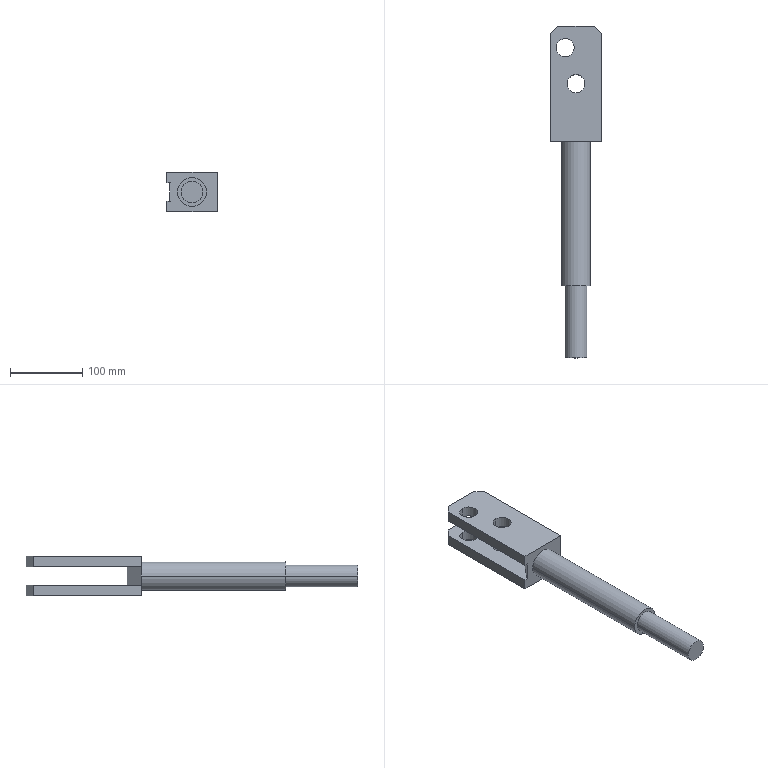Component | SolidWorks | Right-handTieRod1-1 | 1 solid | 30 faces | box 70 x 460 x 55 mm | volume 654381 mm3 | plane 18 | cylinder 12 | commonest cylinder face diameters 25 x8 30 x2 40 x2 | material N/A
build123d program:
from build123d import *

# Parameters (mm, degrees)
BOSS_EXTRUDE1_DEPTH      = 35
SKETCH2_R                = 12.5
CUT_EXTRUDE1_DEPTH       = 60
CHAMFER1_SIZE            = 10
SKETCH3_R                = 20
BOSS_EXTRUDE2_DEPTH      = 300
CHAMFER2_SIZE            = 5
CHAMFER2_SIZE2           = 8.66
SKETCH4_OUTSIDE_W        = 165.706
SKETCH4_OUTSIDE_H        = 150.706
SKETCH4_OUTSIDE_R        = 15
CUT_EXTRUDE2_DEPTH       = 100
CLEVISRELIEF_CRANK_DEPTH = 12.5


with BuildPart() as part:
    # Sketch1 → Boss-Extrude1 (new, symmetric)
    with BuildSketch(Plane(origin=(0, 0, 0), x_dir=(0, 0, -1), z_dir=(1, 0, 0))):
        Polygon((80, 12.5), (-60, 12.5), (-60, -12.5), (80, -12.5), (80, -27.5), (-80, -27.5), (-80, 27.5), (80, 27.5), align=None)
    extrude(amount=BOSS_EXTRUDE1_DEPTH, both=True)

    # Sketch2 → Cut-Extrude1 (cut)
    with BuildSketch(Plane.XZ.offset(27.5)):
        with Locations(Location((-15, -50, 0), (0, 0, 270))):
            Circle(SKETCH2_R)
        with Locations(Location((0, 0, 0), (0, 0, 270))):
            Circle(SKETCH2_R)
    extrude(amount=-CUT_EXTRUDE1_DEPTH, mode=Mode.SUBTRACT)

    # Chamfer1
    chamfer1_edges = [part.edges().sort_by_distance(p)[0] for p in [
        (-35, 20, -80),
        (35, -20, -80),
        (35, 20, -80),
        (-35, -20, -80),
    ]]
    chamfer(chamfer1_edges, length=CHAMFER1_SIZE)

    # Sketch3 → Boss-Extrude2 (add)
    with BuildSketch(Plane.XY.offset(80)):
        Circle(SKETCH3_R)
    extrude(amount=BOSS_EXTRUDE2_DEPTH)

    # Chamfer2
    chamfer2_edges = [part.edges().sort_by_distance(p)[0] for p in [
        (-35, 0, 60),
    ]]
    chamfer2_side = [part.faces().sort_by_distance(p)[0] for p in [
        (-35, 14.098, -5),
    ]]
    chamfer(chamfer2_edges, length=CHAMFER2_SIZE, length2=CHAMFER2_SIZE2, reference=chamfer2_side[0])

    # Sketch4 outside → Cut-Extrude2 (cut)
    with BuildSketch(Plane.XY.offset(380)):
        Rectangle(SKETCH4_OUTSIDE_W, SKETCH4_OUTSIDE_H)
        Circle(SKETCH4_OUTSIDE_R, mode=Mode.SUBTRACT)
    extrude(amount=-CUT_EXTRUDE2_DEPTH, mode=Mode.SUBTRACT)

    # ClevisRelief_Sketch → ClevisRelief_Crank (cut, symmetric)
    with BuildSketch(Plane(origin=(0, 0, 0), x_dir=(1, 0, 0), z_dir=(0, 1, 0))):
        Polygon((-11.942, -57), (-33.339, -83), (-40, -83), (-40, -57), align=None)
    extrude(amount=CLEVISRELIEF_CRANK_DEPTH, both=True, mode=Mode.SUBTRACT)


solid = part.part

# Placed as in the assembly
solid = solid.moved(Location((69.344, 1052.787, 17), (90, 0, 0)))
STEP:
#1=COLOUR_RGB('',0.7922,0.8196,0.9333);
#2=FILL_AREA_STYLE_COLOUR('',#1);
#3=FILL_AREA_STYLE('',(#2));
#4=SURFACE_STYLE_FILL_AREA(#3);
#5=SURFACE_SIDE_STYLE('',(#4));
#6=SURFACE_STYLE_USAGE(.BOTH.,#5);
#7=PRESENTATION_STYLE_ASSIGNMENT((#6));
#8=CARTESIAN_POINT('',(3.321,30.425,0.6693));
#9=VERTEX_POINT('',#8);
#10=CARTESIAN_POINT('',(2.14,30.425,0.6693));
#11=VERTEX_POINT('',#10);
#12=CARTESIAN_POINT('',(2.73,30.425,0.6693));
#13=DIRECTION('',(-0.,-1.,-0.));
#14=DIRECTION('',(1.,0.,0.));
#15=AXIS2_PLACEMENT_3D('',#12,#13,#14);
#16=CIRCLE('',#15,0.5906);
#17=EDGE_CURVE('',#9,#11,#16,.T.);
#18=ORIENTED_EDGE('',*,*,#17,.T.);
#19=CARTESIAN_POINT('',(2.14,26.488,0.6693));
#20=VERTEX_POINT('',#19);
#21=CARTESIAN_POINT('',(2.14,30.425,0.6693));
#22=DIRECTION('',(-0.,-1.,-0.));
#23=VECTOR('',#22,39.37);
#24=LINE('',#21,#23);
#25=EDGE_CURVE('',#11,#20,#24,.T.);
#26=ORIENTED_EDGE('',*,*,#25,.T.);
#27=CARTESIAN_POINT('',(3.321,26.488,0.6693));
#28=VERTEX_POINT('',#27);
#29=CARTESIAN_POINT('',(2.73,26.488,0.6693));
#30=DIRECTION('',(-0.,-1.,-0.));
#31=DIRECTION('',(1.,0.,0.));
#32=AXIS2_PLACEMENT_3D('',#29,#30,#31);
#33=CIRCLE('',#32,0.5906);
#34=EDGE_CURVE('',#28,#20,#33,.T.);
#35=ORIENTED_EDGE('',*,*,#34,.F.);
#36=CARTESIAN_POINT('',(3.321,30.425,0.6693));
#37=DIRECTION('',(-0.,-1.,-0.));
#38=VECTOR('',#37,39.37);
#39=LINE('',#36,#38);
#40=EDGE_CURVE('',#9,#28,#39,.T.);
#41=ORIENTED_EDGE('',*,*,#40,.F.);
#42=EDGE_LOOP('',(#18,#26,#35,#41));
#43=FACE_OUTER_BOUND('',#42,.T.);
#44=CARTESIAN_POINT('',(2.73,30.425,0.6693));
#45=DIRECTION('',(-0.,-1.,-0.));
#46=DIRECTION('',(1.,0.,0.));
#47=AXIS2_PLACEMENT_3D('',#44,#45,#46);
#48=CYLINDRICAL_SURFACE('',#47,0.5906);
#49=ADVANCED_FACE('',(#43),#48,.T.);
#50=CARTESIAN_POINT('',(2.14,42.925,0.1772));
#51=VERTEX_POINT('',#50);
#52=CARTESIAN_POINT('',(2.14,43.909,0.1772));
#53=VERTEX_POINT('',#52);
#54=CARTESIAN_POINT('',(2.14,43.417,0.1772));
#55=DIRECTION('',(-0.,0.,-1.));
#56=DIRECTION('',(0.,1.,0.));
#57=AXIS2_PLACEMENT_3D('',#54,#55,#56);
#58=CIRCLE('',#57,0.4921);
#59=EDGE_CURVE('',#51,#53,#58,.T.);
#60=ORIENTED_EDGE('',*,*,#59,.F.);
#61=CARTESIAN_POINT('',(2.14,42.925,-0.4134));
#62=VERTEX_POINT('',#61);
#63=CARTESIAN_POINT('',(2.14,42.925,1.949));
#64=DIRECTION('',(-0.,0.,-1.));
#65=VECTOR('',#64,39.37);
#66=LINE('',#63,#65);
#67=EDGE_CURVE('',#51,#62,#66,.T.);
#68=ORIENTED_EDGE('',*,*,#67,.T.);
#69=CARTESIAN_POINT('',(2.14,43.909,-0.4134));
#70=VERTEX_POINT('',#69);
#71=CARTESIAN_POINT('',(2.14,43.417,-0.4134));
#72=DIRECTION('',(-0.,0.,-1.));
#73=DIRECTION('',(0.,1.,0.));
#74=AXIS2_PLACEMENT_3D('',#71,#72,#73);
#75=CIRCLE('',#74,0.4921);
#76=EDGE_CURVE('',#62,#70,#75,.T.);
#77=ORIENTED_EDGE('',*,*,#76,.T.);
#78=CARTESIAN_POINT('',(2.14,43.909,1.949));
#79=DIRECTION('',(-0.,0.,-1.));
#80=VECTOR('',#79,39.37);
#81=LINE('',#78,#80);
#82=EDGE_CURVE('',#53,#70,#81,.T.);
#83=ORIENTED_EDGE('',*,*,#82,.F.);
#84=EDGE_LOOP('',(#60,#68,#77,#83));
#85=FACE_OUTER_BOUND('',#84,.T.);
#86=CARTESIAN_POINT('',(2.14,43.417,1.949));
#87=DIRECTION('',(-0.,0.,-1.));
#88=DIRECTION('',(0.,1.,0.));
#89=AXIS2_PLACEMENT_3D('',#86,#87,#88);
#90=CYLINDRICAL_SURFACE('',#89,0.4921);
#91=ADVANCED_FACE('',(#85),#90,.F.);
#92=CARTESIAN_POINT('',(2.73,40.956,0.1772));
#93=VERTEX_POINT('',#92);
#94=CARTESIAN_POINT('',(2.73,41.94,0.1772));
#95=VERTEX_POINT('',#94);
#96=CARTESIAN_POINT('',(2.73,41.448,0.1772));
#97=DIRECTION('',(-0.,0.,-1.));
#98=DIRECTION('',(0.,1.,0.));
#99=AXIS2_PLACEMENT_3D('',#96,#97,#98);
#100=CIRCLE('',#99,0.4921);
#101=EDGE_CURVE('',#93,#95,#100,.T.);
#102=ORIENTED_EDGE('',*,*,#101,.F.);
#103=CARTESIAN_POINT('',(2.73,40.956,-0.4134));
#104=VERTEX_POINT('',#103);
#105=CARTESIAN_POINT('',(2.73,40.956,1.949));
#106=DIRECTION('',(-0.,0.,-1.));
#107=VECTOR('',#106,39.37);
#108=LINE('',#105,#107);
#109=EDGE_CURVE('',#93,#104,#108,.T.);
#110=ORIENTED_EDGE('',*,*,#109,.T.);
#111=CARTESIAN_POINT('',(2.73,41.94,-0.4134));
#112=VERTEX_POINT('',#111);
#113=CARTESIAN_POINT('',(2.73,41.448,-0.4134));
#114=DIRECTION('',(-0.,0.,-1.));
#115=DIRECTION('',(0.,1.,0.));
#116=AXIS2_PLACEMENT_3D('',#113,#114,#115);
#117=CIRCLE('',#116,0.4921);
#118=EDGE_CURVE('',#104,#112,#117,.T.);
#119=ORIENTED_EDGE('',*,*,#118,.T.);
#120=CARTESIAN_POINT('',(2.73,41.94,1.949));
#121=DIRECTION('',(-0.,0.,-1.));
#122=VECTOR('',#121,39.37);
#123=LINE('',#120,#122);
#124=EDGE_CURVE('',#95,#112,#123,.T.);
#125=ORIENTED_EDGE('',*,*,#124,.F.);
#126=EDGE_LOOP('',(#102,#110,#119,#125));
#127=FACE_OUTER_BOUND('',#126,.T.);
#128=CARTESIAN_POINT('',(2.73,41.448,1.949));
#129=DIRECTION('',(-0.,0.,-1.));
#130=DIRECTION('',(0.,1.,0.));
#131=AXIS2_PLACEMENT_3D('',#128,#129,#130);
#132=CYLINDRICAL_SURFACE('',#131,0.4921);
#133=ADVANCED_FACE('',(#127),#132,.F.);
#134=CARTESIAN_POINT('',(2.14,42.925,1.752));
#135=VERTEX_POINT('',#134);
#136=CARTESIAN_POINT('',(2.14,43.909,1.752));
#137=VERTEX_POINT('',#136);
#138=CARTESIAN_POINT('',(2.14,43.417,1.752));
#139=DIRECTION('',(-0.,0.,-1.));
#140=DIRECTION('',(0.,1.,0.));
#141=AXIS2_PLACEMENT_3D('',#138,#139,#140);
#142=CIRCLE('',#141,0.4921);
#143=EDGE_CURVE('',#135,#137,#142,.T.);
#144=ORIENTED_EDGE('',*,*,#143,.F.);
#145=CARTESIAN_POINT('',(2.14,42.925,1.161));
#146=VERTEX_POINT('',#145);
#147=CARTESIAN_POINT('',(2.14,42.925,1.949));
#148=DIRECTION('',(-0.,0.,-1.));
#149=VECTOR('',#148,39.37);
#150=LINE('',#147,#149);
#151=EDGE_CURVE('',#135,#146,#150,.T.);
#152=ORIENTED_EDGE('',*,*,#151,.T.);
#153=CARTESIAN_POINT('',(2.14,43.909,1.161));
#154=VERTEX_POINT('',#153);
#155=CARTESIAN_POINT('',(2.14,43.417,1.161));
#156=DIRECTION('',(0.,-0.,1.));
#157=DIRECTION('',(-0.,-1.,-0.));
#158=AXIS2_PLACEMENT_3D('',#155,#156,#157);
#159=CIRCLE('',#158,0.4921);
#160=EDGE_CURVE('',#154,#146,#159,.T.);
#161=ORIENTED_EDGE('',*,*,#160,.F.);
#162=CARTESIAN_POINT('',(2.14,43.909,1.949));
#163=DIRECTION('',(-0.,0.,-1.));
#164=VECTOR('',#163,39.37);
#165=LINE('',#162,#164);
#166=EDGE_CURVE('',#137,#154,#165,.T.);
#167=ORIENTED_EDGE('',*,*,#166,.F.);
#168=EDGE_LOOP('',(#144,#152,#161,#167));
#169=FACE_OUTER_BOUND('',#168,.T.);
#170=CARTESIAN_POINT('',(2.14,43.417,1.949));
#171=DIRECTION('',(-0.,0.,-1.));
#172=DIRECTION('',(0.,1.,0.));
#173=AXIS2_PLACEMENT_3D('',#170,#171,#172);
#174=CYLINDRICAL_SURFACE('',#173,0.4921);
#175=ADVANCED_FACE('',(#169),#174,.F.);
#176=CARTESIAN_POINT('',(2.73,40.956,1.752));
#177=VERTEX_POINT('',#176);
#178=CARTESIAN_POINT('',(2.73,41.94,1.752));
#179=VERTEX_POINT('',#178);
#180=CARTESIAN_POINT('',(2.73,41.448,1.752));
#181=DIRECTION('',(-0.,0.,-1.));
#182=DIRECTION('',(0.,1.,0.));
#183=AXIS2_PLACEMENT_3D('',#180,#181,#182);
#184=CIRCLE('',#183,0.4921);
#185=EDGE_CURVE('',#177,#179,#184,.T.);
#186=ORIENTED_EDGE('',*,*,#185,.F.);
#187=CARTESIAN_POINT('',(2.73,40.956,1.161));
#188=VERTEX_POINT('',#187);
#189=CARTESIAN_POINT('',(2.73,40.956,1.949));
#190=DIRECTION('',(-0.,0.,-1.));
#191=VECTOR('',#190,39.37);
#192=LINE('',#189,#191);
#193=EDGE_CURVE('',#177,#188,#192,.T.);
#194=ORIENTED_EDGE('',*,*,#193,.T.);
#195=CARTESIAN_POINT('',(2.73,41.94,1.161));
#196=VERTEX_POINT('',#195);
#197=CARTESIAN_POINT('',(2.73,41.448,1.161));
#198=DIRECTION('',(0.,-0.,1.));
#199=DIRECTION('',(-0.,-1.,-0.));
#200=AXIS2_PLACEMENT_3D('',#197,#198,#199);
#201=CIRCLE('',#200,0.4921);
#202=EDGE_CURVE('',#196,#188,#201,.T.);
#203=ORIENTED_EDGE('',*,*,#202,.F.);
#204=CARTESIAN_POINT('',(2.73,41.94,1.949));
#205=DIRECTION('',(-0.,0.,-1.));
#206=VECTOR('',#205,39.37);
#207=LINE('',#204,#206);
#208=EDGE_CURVE('',#179,#196,#207,.T.);
#209=ORIENTED_EDGE('',*,*,#208,.F.);
#210=EDGE_LOOP('',(#186,#194,#203,#209));
#211=FACE_OUTER_BOUND('',#210,.T.);
#212=CARTESIAN_POINT('',(2.73,41.448,1.949));
#213=DIRECTION('',(-0.,0.,-1.));
#214=DIRECTION('',(0.,1.,0.));
#215=AXIS2_PLACEMENT_3D('',#212,#213,#214);
#216=CYLINDRICAL_SURFACE('',#215,0.4921);
#217=ADVANCED_FACE('',(#211),#216,.F.);
#218=CARTESIAN_POINT('',(3.517,30.425,0.6693));
#219=VERTEX_POINT('',#218);
#220=CARTESIAN_POINT('',(1.943,30.425,0.6693));
#221=VERTEX_POINT('',#220);
#222=CARTESIAN_POINT('',(2.73,30.425,0.6693));
#223=DIRECTION('',(-0.,-1.,-0.));
#224=DIRECTION('',(1.,0.,0.));
#225=AXIS2_PLACEMENT_3D('',#222,#223,#224);
#226=CIRCLE('',#225,0.7874);
#227=EDGE_CURVE('',#219,#221,#226,.T.);
#228=ORIENTED_EDGE('',*,*,#227,.F.);
#229=CARTESIAN_POINT('',(3.517,38.299,0.6693));
#230=VERTEX_POINT('',#229);
#231=CARTESIAN_POINT('',(3.517,26.488,0.6693));
#232=DIRECTION('',(0.,1.,0.));
#233=VECTOR('',#232,39.37);
#234=LINE('',#231,#233);
#235=EDGE_CURVE('',#219,#230,#234,.T.);
#236=ORIENTED_EDGE('',*,*,#235,.T.);
#237=CARTESIAN_POINT('',(1.943,38.299,0.6693));
#238=VERTEX_POINT('',#237);
#239=CARTESIAN_POINT('',(2.73,38.299,0.6693));
#240=DIRECTION('',(-0.,-1.,-0.));
#241=DIRECTION('',(1.,0.,0.));
#242=AXIS2_PLACEMENT_3D('',#239,#240,#241);
#243=CIRCLE('',#242,0.7874);
#244=EDGE_CURVE('',#230,#238,#243,.T.);
#245=ORIENTED_EDGE('',*,*,#244,.T.);
#246=CARTESIAN_POINT('',(1.943,26.488,0.6693));
#247=DIRECTION('',(0.,1.,0.));
#248=VECTOR('',#247,39.37);
#249=LINE('',#246,#248);
#250=EDGE_CURVE('',#221,#238,#249,.T.);
#251=ORIENTED_EDGE('',*,*,#250,.F.);
#252=EDGE_LOOP('',(#228,#236,#245,#251));
#253=FACE_OUTER_BOUND('',#252,.T.);
#254=CARTESIAN_POINT('',(2.73,26.488,0.6693));
#255=DIRECTION('',(0.,1.,0.));
#256=DIRECTION('',(-1.,0.,0.));
#257=AXIS2_PLACEMENT_3D('',#254,#255,#256);
#258=CYLINDRICAL_SURFACE('',#257,0.7874);
#259=ADVANCED_FACE('',(#253),#258,.T.);
#260=CARTESIAN_POINT('',(2.73,38.299,0.6693));
#261=DIRECTION('',(-0.,-1.,-0.));
#262=DIRECTION('',(1.,0.,0.));
#263=AXIS2_PLACEMENT_3D('',#260,#261,#262);
#264=CIRCLE('',#263,0.7874);
#265=EDGE_CURVE('',#238,#230,#264,.T.);
#266=ORIENTED_EDGE('',*,*,#265,.F.);
#267=ORIENTED_EDGE('',*,*,#244,.F.);
#268=EDGE_LOOP('',(#266,#267));
#269=FACE_BOUND('',#268,.T.);
#270=CARTESIAN_POINT('',(1.352,38.299,0.1772));
#271=VERTEX_POINT('',#270);
#272=CARTESIAN_POINT('',(1.515,38.299,0.1772));
#273=VERTEX_POINT('',#272);
#274=CARTESIAN_POINT('',(4.108,38.299,0.1772));
#275=DIRECTION('',(1.,-0.,-0.));
#276=VECTOR('',#275,39.37);
#277=LINE('',#274,#276);
#278=EDGE_CURVE('',#271,#273,#277,.T.);
#279=ORIENTED_EDGE('',*,*,#278,.F.);
#280=CARTESIAN_POINT('',(1.352,38.299,-0.4134));
#281=VERTEX_POINT('',#280);
#282=CARTESIAN_POINT('',(1.352,38.299,-0.4134));
#283=DIRECTION('',(-0.,-0.,-1.));
#284=VECTOR('',#283,39.37);
#285=LINE('',#282,#284);
#286=EDGE_CURVE('',#271,#281,#285,.T.);
#287=ORIENTED_EDGE('',*,*,#286,.T.);
#288=CARTESIAN_POINT('',(4.108,38.299,-0.4134));
#289=VERTEX_POINT('',#288);
#290=CARTESIAN_POINT('',(4.108,38.299,-0.4134));
#291=DIRECTION('',(-1.,0.,0.));
#292=VECTOR('',#291,39.37);
#293=LINE('',#290,#292);
#294=EDGE_CURVE('',#289,#281,#293,.T.);
#295=ORIENTED_EDGE('',*,*,#294,.F.);
#296=CARTESIAN_POINT('',(4.108,38.299,1.752));
#297=VERTEX_POINT('',#296);
#298=CARTESIAN_POINT('',(4.108,38.299,-0.4134));
#299=DIRECTION('',(-0.,-0.,-1.));
#300=VECTOR('',#299,39.37);
#301=LINE('',#298,#300);
#302=EDGE_CURVE('',#297,#289,#301,.T.);
#303=ORIENTED_EDGE('',*,*,#302,.F.);
#304=CARTESIAN_POINT('',(1.352,38.299,1.752));
#305=VERTEX_POINT('',#304);
#306=CARTESIAN_POINT('',(4.108,38.299,1.752));
#307=DIRECTION('',(-1.,0.,0.));
#308=VECTOR('',#307,39.37);
#309=LINE('',#306,#308);
#310=EDGE_CURVE('',#297,#305,#309,.T.);
#311=ORIENTED_EDGE('',*,*,#310,.T.);
#312=CARTESIAN_POINT('',(1.352,38.299,1.161));
#313=VERTEX_POINT('',#312);
#314=CARTESIAN_POINT('',(1.352,38.299,-0.4134));
#315=DIRECTION('',(-0.,-0.,-1.));
#316=VECTOR('',#315,39.37);
#317=LINE('',#314,#316);
#318=EDGE_CURVE('',#305,#313,#317,.T.);
#319=ORIENTED_EDGE('',*,*,#318,.T.);
#320=CARTESIAN_POINT('',(1.515,38.299,1.161));
#321=VERTEX_POINT('',#320);
#322=CARTESIAN_POINT('',(4.108,38.299,1.161));
#323=DIRECTION('',(1.,-0.,-0.));
#324=VECTOR('',#323,39.37);
#325=LINE('',#322,#324);
#326=EDGE_CURVE('',#313,#321,#325,.T.);
#327=ORIENTED_EDGE('',*,*,#326,.T.);
#328=CARTESIAN_POINT('',(1.515,38.299,-0.4134));
#329=DIRECTION('',(-0.,-0.,-1.));
#330=VECTOR('',#329,39.37);
#331=LINE('',#328,#330);
#332=EDGE_CURVE('',#321,#273,#331,.T.);
#333=ORIENTED_EDGE('',*,*,#332,.T.);
#334=EDGE_LOOP('',(#279,#287,#295,#303,#311,#319,#327,#333));
#335=FACE_OUTER_BOUND('',#334,.T.);
#336=CARTESIAN_POINT('',(4.108,38.299,-0.4134));
#337=DIRECTION('',(0.,1.,-0.));
#338=DIRECTION('',(0.,0.,1.));
#339=AXIS2_PLACEMENT_3D('',#336,#337,#338);
#340=PLANE('',#339);
#341=ADVANCED_FACE('',(#269,#335),#340,.F.);
#342=ORIENTED_EDGE('',*,*,#286,.F.);
#343=CARTESIAN_POINT('',(1.352,44.204,0.1772));
#344=VERTEX_POINT('',#343);
#345=CARTESIAN_POINT('',(1.352,39.086,0.1772));
#346=DIRECTION('',(-0.,-1.,-0.));
#347=VECTOR('',#346,39.37);
#348=LINE('',#345,#347);
#349=EDGE_CURVE('',#344,#271,#348,.T.);
#350=ORIENTED_EDGE('',*,*,#349,.F.);
#351=CARTESIAN_POINT('',(1.352,44.204,-0.4134));
#352=VERTEX_POINT('',#351);
#353=CARTESIAN_POINT('',(1.352,44.204,-0.4134));
#354=DIRECTION('',(-0.,-0.,-1.));
#355=VECTOR('',#354,39.37);
#356=LINE('',#353,#355);
#357=EDGE_CURVE('',#344,#352,#356,.T.);
#358=ORIENTED_EDGE('',*,*,#357,.T.);
#359=CARTESIAN_POINT('',(1.352,38.299,-0.4134));
#360=DIRECTION('',(0.,1.,-0.));
#361=VECTOR('',#360,39.37);
#362=LINE('',#359,#361);
#363=EDGE_CURVE('',#281,#352,#362,.T.);
#364=ORIENTED_EDGE('',*,*,#363,.F.);
#365=EDGE_LOOP('',(#342,#350,#358,#364));
#366=FACE_OUTER_BOUND('',#365,.T.);
#367=CARTESIAN_POINT('',(1.352,41.448,0.6693));
#368=DIRECTION('',(-1.,0.,0.));
#369=DIRECTION('',(-0.,-1.,-0.));
#370=AXIS2_PLACEMENT_3D('',#367,#368,#369);
#371=PLANE('',#370);
#372=ADVANCED_FACE('',(#366),#371,.T.);
#373=ORIENTED_EDGE('',*,*,#235,.F.);
#374=CARTESIAN_POINT('',(2.73,30.425,0.6693));
#375=DIRECTION('',(-0.,-1.,-0.));
#376=DIRECTION('',(1.,0.,0.));
#377=AXIS2_PLACEMENT_3D('',#374,#375,#376);
#378=CIRCLE('',#377,0.7874);
#379=EDGE_CURVE('',#221,#219,#378,.T.);
#380=ORIENTED_EDGE('',*,*,#379,.F.);
#381=ORIENTED_EDGE('',*,*,#250,.T.);
#382=ORIENTED_EDGE('',*,*,#265,.T.);
#383=EDGE_LOOP('',(#373,#380,#381,#382));
#384=FACE_OUTER_BOUND('',#383,.T.);
#385=CARTESIAN_POINT('',(2.73,26.488,0.6693));
#386=DIRECTION('',(0.,1.,0.));
#387=DIRECTION('',(-1.,0.,0.));
#388=AXIS2_PLACEMENT_3D('',#385,#386,#387);
#389=CYLINDRICAL_SURFACE('',#388,0.7874);
#390=ADVANCED_FACE('',(#384),#389,.T.);
#391=CARTESIAN_POINT('',(3.714,44.598,1.161));
#392=VERTEX_POINT('',#391);
#393=CARTESIAN_POINT('',(1.746,44.598,1.161));
#394=VERTEX_POINT('',#393);
#395=CARTESIAN_POINT('',(4.108,44.598,1.161));
#396=DIRECTION('',(-1.,0.,0.));
#397=VECTOR('',#396,39.37);
#398=LINE('',#395,#397);
#399=EDGE_CURVE('',#392,#394,#398,.T.);
#400=ORIENTED_EDGE('',*,*,#399,.T.);
#401=CARTESIAN_POINT('',(1.746,44.598,1.752));
#402=VERTEX_POINT('',#401);
#403=CARTESIAN_POINT('',(1.746,44.598,1.752));
#404=DIRECTION('',(0.,-0.,1.));
#405=VECTOR('',#404,39.37);
#406=LINE('',#403,#405);
#407=EDGE_CURVE('',#394,#402,#406,.T.);
#408=ORIENTED_EDGE('',*,*,#407,.T.);
#409=CARTESIAN_POINT('',(3.714,44.598,1.752));
#410=VERTEX_POINT('',#409);
#411=CARTESIAN_POINT('',(4.108,44.598,1.752));
#412=DIRECTION('',(-1.,0.,0.));
#413=VECTOR('',#412,39.37);
#414=LINE('',#411,#413);
#415=EDGE_CURVE('',#410,#402,#414,.T.);
#416=ORIENTED_EDGE('',*,*,#415,.F.);
#417=CARTESIAN_POINT('',(3.714,44.598,1.161));
#418=DIRECTION('',(-0.,0.,-1.));
#419=VECTOR('',#418,39.37);
#420=LINE('',#417,#419);
#421=EDGE_CURVE('',#410,#392,#420,.T.);
#422=ORIENTED_EDGE('',*,*,#421,.T.);
#423=EDGE_LOOP('',(#400,#408,#416,#422));
#424=FACE_OUTER_BOUND('',#423,.T.);
#425=CARTESIAN_POINT('',(4.108,44.598,1.161));
#426=DIRECTION('',(-0.,-1.,-0.));
#427=DIRECTION('',(-0.,0.,-1.));
#428=AXIS2_PLACEMENT_3D('',#425,#426,#427);
#429=PLANE('',#428);
#430=ADVANCED_FACE('',(#424),#429,.F.);
#431=CARTESIAN_POINT('',(2.14,43.417,1.752));
#432=DIRECTION('',(-0.,0.,-1.));
#433=DIRECTION('',(0.,1.,0.));
#434=AXIS2_PLACEMENT_3D('',#431,#432,#433);
#435=CIRCLE('',#434,0.4921);
#436=EDGE_CURVE('',#137,#135,#435,.T.);
#437=ORIENTED_EDGE('',*,*,#436,.T.);
#438=ORIENTED_EDGE('',*,*,#143,.T.);
#439=EDGE_LOOP('',(#437,#438));
#440=FACE_BOUND('',#439,.T.);
#441=CARTESIAN_POINT('',(2.73,41.448,1.752));
#442=DIRECTION('',(-0.,0.,-1.));
#443=DIRECTION('',(0.,1.,0.));
#444=AXIS2_PLACEMENT_3D('',#441,#442,#443);
#445=CIRCLE('',#444,0.4921);
#446=EDGE_CURVE('',#179,#177,#445,.T.);
#447=ORIENTED_EDGE('',*,*,#446,.T.);
#448=ORIENTED_EDGE('',*,*,#185,.T.);
#449=EDGE_LOOP('',(#447,#448));
#450=FACE_BOUND('',#449,.T.);
#451=ORIENTED_EDGE('',*,*,#415,.T.);
#452=CARTESIAN_POINT('',(1.352,44.204,1.752));
#453=VERTEX_POINT('',#452);
#454=CARTESIAN_POINT('',(1.746,44.598,1.752));
#455=DIRECTION('',(-0.7071,-0.7071,-0.));
#456=VECTOR('',#455,39.37);
#457=LINE('',#454,#456);
#458=EDGE_CURVE('',#402,#453,#457,.T.);
#459=ORIENTED_EDGE('',*,*,#458,.T.);
#460=CARTESIAN_POINT('',(1.352,38.299,1.752));
#461=DIRECTION('',(-0.,-1.,-0.));
#462=VECTOR('',#461,39.37);
#463=LINE('',#460,#462);
#464=EDGE_CURVE('',#453,#305,#463,.T.);
#465=ORIENTED_EDGE('',*,*,#464,.T.);
#466=ORIENTED_EDGE('',*,*,#310,.F.);
#467=CARTESIAN_POINT('',(4.108,44.204,1.752));
#468=VERTEX_POINT('',#467);
#469=CARTESIAN_POINT('',(4.108,38.299,1.752));
#470=DIRECTION('',(-0.,-1.,-0.));
#471=VECTOR('',#470,39.37);
#472=LINE('',#469,#471);
#473=EDGE_CURVE('',#468,#297,#472,.T.);
#474=ORIENTED_EDGE('',*,*,#473,.F.);
#475=CARTESIAN_POINT('',(4.108,44.204,1.752));
#476=DIRECTION('',(-0.7071,0.7071,0.));
#477=VECTOR('',#476,39.37);
#478=LINE('',#475,#477);
#479=EDGE_CURVE('',#468,#410,#478,.T.);
#480=ORIENTED_EDGE('',*,*,#479,.T.);
#481=EDGE_LOOP('',(#451,#459,#465,#466,#474,#480));
#482=FACE_OUTER_BOUND('',#481,.T.);
#483=CARTESIAN_POINT('',(4.108,38.299,1.752));
#484=DIRECTION('',(-0.,0.,-1.));
#485=DIRECTION('',(0.,1.,0.));
#486=AXIS2_PLACEMENT_3D('',#483,#484,#485);
#487=PLANE('',#486);
#488=ADVANCED_FACE('',(#440,#450,#482),#487,.F.);
#489=CARTESIAN_POINT('',(2.14,43.417,-0.4134));
#490=DIRECTION('',(-0.,0.,-1.));
#491=DIRECTION('',(0.,1.,0.));
#492=AXIS2_PLACEMENT_3D('',#489,#490,#491);
#493=CIRCLE('',#492,0.4921);
#494=EDGE_CURVE('',#70,#62,#493,.T.);
#495=ORIENTED_EDGE('',*,*,#494,.F.);
#496=ORIENTED_EDGE('',*,*,#76,.F.);
#497=EDGE_LOOP('',(#495,#496));
#498=FACE_BOUND('',#497,.T.);
#499=CARTESIAN_POINT('',(2.73,41.448,-0.4134));
#500=DIRECTION('',(-0.,0.,-1.));
#501=DIRECTION('',(0.,1.,0.));
#502=AXIS2_PLACEMENT_3D('',#499,#500,#501);
#503=CIRCLE('',#502,0.4921);
#504=EDGE_CURVE('',#112,#104,#503,.T.);
#505=ORIENTED_EDGE('',*,*,#504,.F.);
#506=ORIENTED_EDGE('',*,*,#118,.F.);
#507=EDGE_LOOP('',(#505,#506));
#508=FACE_BOUND('',#507,.T.);
#509=ORIENTED_EDGE('',*,*,#363,.T.);
#510=CARTESIAN_POINT('',(1.746,44.598,-0.4134));
#511=VERTEX_POINT('',#510);
#512=CARTESIAN_POINT('',(1.746,44.598,-0.4134));
#513=DIRECTION('',(0.7071,0.7071,-0.));
#514=VECTOR('',#513,39.37);
#515=LINE('',#512,#514);
#516=EDGE_CURVE('',#352,#511,#515,.T.);
#517=ORIENTED_EDGE('',*,*,#516,.T.);
#518=CARTESIAN_POINT('',(3.714,44.598,-0.4134));
#519=VERTEX_POINT('',#518);
#520=CARTESIAN_POINT('',(4.108,44.598,-0.4134));
#521=DIRECTION('',(-1.,0.,0.));
#522=VECTOR('',#521,39.37);
#523=LINE('',#520,#522);
#524=EDGE_CURVE('',#519,#511,#523,.T.);
#525=ORIENTED_EDGE('',*,*,#524,.F.);
#526=CARTESIAN_POINT('',(4.108,44.204,-0.4134));
#527=VERTEX_POINT('',#526);
#528=CARTESIAN_POINT('',(4.108,44.204,-0.4134));
#529=DIRECTION('',(0.7071,-0.7071,0.));
#530=VECTOR('',#529,39.37);
#531=LINE('',#528,#530);
#532=EDGE_CURVE('',#519,#527,#531,.T.);
#533=ORIENTED_EDGE('',*,*,#532,.T.);
#534=CARTESIAN_POINT('',(4.108,38.299,-0.4134));
#535=DIRECTION('',(0.,1.,-0.));
#536=VECTOR('',#535,39.37);
#537=LINE('',#534,#536);
#538=EDGE_CURVE('',#289,#527,#537,.T.);
#539=ORIENTED_EDGE('',*,*,#538,.F.);
#540=ORIENTED_EDGE('',*,*,#294,.T.);
#541=EDGE_LOOP('',(#509,#517,#525,#533,#539,#540));
#542=FACE_OUTER_BOUND('',#541,.T.);
#543=CARTESIAN_POINT('',(4.108,38.299,-0.4134));
#544=DIRECTION('',(0.,0.,1.));
#545=DIRECTION('',(-0.,-1.,0.));
#546=AXIS2_PLACEMENT_3D('',#543,#544,#545);
#547=PLANE('',#546);
#548=ADVANCED_FACE('',(#498,#508,#542),#547,.F.);
#549=ORIENTED_EDGE('',*,*,#524,.T.);
#550=CARTESIAN_POINT('',(1.746,44.598,0.1772));
#551=VERTEX_POINT('',#550);
#552=CARTESIAN_POINT('',(1.746,44.598,0.1772));
#553=DIRECTION('',(0.,0.,1.));
#554=VECTOR('',#553,39.37);
#555=LINE('',#552,#554);
#556=EDGE_CURVE('',#511,#551,#555,.T.);
#557=ORIENTED_EDGE('',*,*,#556,.T.);
#558=CARTESIAN_POINT('',(3.714,44.598,0.1772));
#559=VERTEX_POINT('',#558);
#560=CARTESIAN_POINT('',(4.108,44.598,0.1772));
#561=DIRECTION('',(-1.,0.,0.));
#562=VECTOR('',#561,39.37);
#563=LINE('',#560,#562);
#564=EDGE_CURVE('',#559,#551,#563,.T.);
#565=ORIENTED_EDGE('',*,*,#564,.F.);
#566=CARTESIAN_POINT('',(3.714,44.598,-0.4134));
#567=DIRECTION('',(-0.,-0.,-1.));
#568=VECTOR('',#567,39.37);
#569=LINE('',#566,#568);
#570=EDGE_CURVE('',#559,#519,#569,.T.);
#571=ORIENTED_EDGE('',*,*,#570,.T.);
#572=EDGE_LOOP('',(#549,#557,#565,#571));
#573=FACE_OUTER_BOUND('',#572,.T.);
#574=CARTESIAN_POINT('',(4.108,44.598,-0.4134));
#575=DIRECTION('',(-0.,-1.,0.));
#576=DIRECTION('',(-0.,-0.,-1.));
#577=AXIS2_PLACEMENT_3D('',#574,#575,#576);
#578=PLANE('',#577);
#579=ADVANCED_FACE('',(#573),#578,.F.);
#580=ORIENTED_EDGE('',*,*,#349,.T.);
#581=ORIENTED_EDGE('',*,*,#278,.T.);
#582=CARTESIAN_POINT('',(2.163,39.086,0.1772));
#583=VERTEX_POINT('',#582);
#584=CARTESIAN_POINT('',(2.26,39.204,0.1772));
#585=DIRECTION('',(0.6354,0.7721,0.));
#586=VECTOR('',#585,39.37);
#587=LINE('',#584,#586);
#588=EDGE_CURVE('',#273,#583,#587,.T.);
#589=ORIENTED_EDGE('',*,*,#588,.T.);
#590=CARTESIAN_POINT('',(4.108,39.086,0.1772));
#591=VERTEX_POINT('',#590);
#592=CARTESIAN_POINT('',(4.108,39.086,0.1772));
#593=DIRECTION('',(-1.,0.,0.));
#594=VECTOR('',#593,39.37);
#595=LINE('',#592,#594);
#596=EDGE_CURVE('',#591,#583,#595,.T.);
#597=ORIENTED_EDGE('',*,*,#596,.F.);
#598=CARTESIAN_POINT('',(4.108,44.204,0.1772));
#599=VERTEX_POINT('',#598);
#600=CARTESIAN_POINT('',(4.108,39.086,0.1772));
#601=DIRECTION('',(-0.,-1.,-0.));
#602=VECTOR('',#601,39.37);
#603=LINE('',#600,#602);
#604=EDGE_CURVE('',#599,#591,#603,.T.);
#605=ORIENTED_EDGE('',*,*,#604,.F.);
#606=CARTESIAN_POINT('',(4.108,44.204,0.1772));
#607=DIRECTION('',(-0.7071,0.7071,0.));
#608=VECTOR('',#607,39.37);
#609=LINE('',#606,#608);
#610=EDGE_CURVE('',#599,#559,#609,.T.);
#611=ORIENTED_EDGE('',*,*,#610,.T.);
#612=ORIENTED_EDGE('',*,*,#564,.T.);
#613=CARTESIAN_POINT('',(1.746,44.598,0.1772));
#614=DIRECTION('',(-0.7071,-0.7071,-0.));
#615=VECTOR('',#614,39.37);
#616=LINE('',#613,#615);
#617=EDGE_CURVE('',#551,#344,#616,.T.);
#618=ORIENTED_EDGE('',*,*,#617,.T.);
#619=EDGE_LOOP('',(#580,#581,#589,#597,#605,#611,#612,#618));
#620=FACE_OUTER_BOUND('',#619,.T.);
#621=CARTESIAN_POINT('',(2.73,41.448,0.1772));
#622=DIRECTION('',(-0.,0.,-1.));
#623=DIRECTION('',(0.,1.,0.));
#624=AXIS2_PLACEMENT_3D('',#621,#622,#623);
#625=CIRCLE('',#624,0.4921);
#626=EDGE_CURVE('',#95,#93,#625,.T.);
#627=ORIENTED_EDGE('',*,*,#626,.T.);
#628=ORIENTED_EDGE('',*,*,#101,.T.);
#629=EDGE_LOOP('',(#627,#628));
#630=FACE_BOUND('',#629,.T.);
#631=CARTESIAN_POINT('',(2.14,43.417,0.1772));
#632=DIRECTION('',(-0.,0.,-1.));
#633=DIRECTION('',(0.,1.,0.));
#634=AXIS2_PLACEMENT_3D('',#631,#632,#633);
#635=CIRCLE('',#634,0.4921);
#636=EDGE_CURVE('',#53,#51,#635,.T.);
#637=ORIENTED_EDGE('',*,*,#636,.T.);
#638=ORIENTED_EDGE('',*,*,#59,.T.);
#639=EDGE_LOOP('',(#637,#638));
#640=FACE_BOUND('',#639,.T.);
#641=CARTESIAN_POINT('',(4.108,39.086,0.1772));
#642=DIRECTION('',(-0.,0.,-1.));
#643=DIRECTION('',(0.,1.,0.));
#644=AXIS2_PLACEMENT_3D('',#641,#642,#643);
#645=PLANE('',#644);
#646=ADVANCED_FACE('',(#620,#630,#640),#645,.F.);
#647=ORIENTED_EDGE('',*,*,#596,.T.);
#648=CARTESIAN_POINT('',(2.163,39.086,1.161));
#649=VERTEX_POINT('',#648);
#650=CARTESIAN_POINT('',(2.163,39.086,1.161));
#651=DIRECTION('',(0.,-0.,1.));
#652=VECTOR('',#651,39.37);
#653=LINE('',#650,#652);
#654=EDGE_CURVE('',#583,#649,#653,.T.);
#655=ORIENTED_EDGE('',*,*,#654,.T.);
#656=CARTESIAN_POINT('',(4.108,39.086,1.161));
#657=VERTEX_POINT('',#656);
#658=CARTESIAN_POINT('',(4.108,39.086,1.161));
#659=DIRECTION('',(-1.,0.,0.));
#660=VECTOR('',#659,39.37);
#661=LINE('',#658,#660);
#662=EDGE_CURVE('',#657,#649,#661,.T.);
#663=ORIENTED_EDGE('',*,*,#662,.F.);
#664=CARTESIAN_POINT('',(4.108,39.086,1.161));
#665=DIRECTION('',(0.,-0.,1.));
#666=VECTOR('',#665,39.37);
#667=LINE('',#664,#666);
#668=EDGE_CURVE('',#591,#657,#667,.T.);
#669=ORIENTED_EDGE('',*,*,#668,.F.);
#670=EDGE_LOOP('',(#647,#655,#663,#669));
#671=FACE_OUTER_BOUND('',#670,.T.);
#672=CARTESIAN_POINT('',(4.108,39.086,1.161));
#673=DIRECTION('',(-0.,-1.,-0.));
#674=DIRECTION('',(1.,-0.,-0.));
#675=AXIS2_PLACEMENT_3D('',#672,#673,#674);
#676=PLANE('',#675);
#677=ADVANCED_FACE('',(#671),#676,.F.);
#678=CARTESIAN_POINT('',(1.352,44.204,1.161));
#679=VERTEX_POINT('',#678);
#680=CARTESIAN_POINT('',(1.352,44.598,1.161));
#681=DIRECTION('',(0.,1.,0.));
#682=VECTOR('',#681,39.37);
#683=LINE('',#680,#682);
#684=EDGE_CURVE('',#313,#679,#683,.T.);
#685=ORIENTED_EDGE('',*,*,#684,.T.);
#686=CARTESIAN_POINT('',(1.746,44.598,1.161));
#687=DIRECTION('',(0.7071,0.7071,0.));
#688=VECTOR('',#687,39.37);
#689=LINE('',#686,#688);
#690=EDGE_CURVE('',#679,#394,#689,.T.);
#691=ORIENTED_EDGE('',*,*,#690,.T.);
#692=ORIENTED_EDGE('',*,*,#399,.F.);
#693=CARTESIAN_POINT('',(4.108,44.204,1.161));
#694=VERTEX_POINT('',#693);
#695=CARTESIAN_POINT('',(4.108,44.204,1.161));
#696=DIRECTION('',(0.7071,-0.7071,-0.));
#697=VECTOR('',#696,39.37);
#698=LINE('',#695,#697);
#699=EDGE_CURVE('',#392,#694,#698,.T.);
#700=ORIENTED_EDGE('',*,*,#699,.T.);
#701=CARTESIAN_POINT('',(4.108,44.598,1.161));
#702=DIRECTION('',(0.,1.,0.));
#703=VECTOR('',#702,39.37);
#704=LINE('',#701,#703);
#705=EDGE_CURVE('',#657,#694,#704,.T.);
#706=ORIENTED_EDGE('',*,*,#705,.F.);
#707=ORIENTED_EDGE('',*,*,#662,.T.);
#708=CARTESIAN_POINT('',(2.26,39.204,1.161));
#709=DIRECTION('',(0.6354,0.7721,0.));
#710=VECTOR('',#709,39.37);
#711=LINE('',#708,#710);
#712=EDGE_CURVE('',#321,#649,#711,.T.);
#713=ORIENTED_EDGE('',*,*,#712,.F.);
#714=ORIENTED_EDGE('',*,*,#326,.F.);
#715=EDGE_LOOP('',(#685,#691,#692,#700,#706,#707,#713,#714));
#716=FACE_OUTER_BOUND('',#715,.T.);
#717=ORIENTED_EDGE('',*,*,#160,.T.);
#718=CARTESIAN_POINT('',(2.14,43.417,1.161));
#719=DIRECTION('',(0.,-0.,1.));
#720=DIRECTION('',(-0.,-1.,-0.));
#721=AXIS2_PLACEMENT_3D('',#718,#719,#720);
#722=CIRCLE('',#721,0.4921);
#723=EDGE_CURVE('',#146,#154,#722,.T.);
#724=ORIENTED_EDGE('',*,*,#723,.T.);
#725=EDGE_LOOP('',(#717,#724));
#726=FACE_BOUND('',#725,.T.);
#727=ORIENTED_EDGE('',*,*,#202,.T.);
#728=CARTESIAN_POINT('',(2.73,41.448,1.161));
#729=DIRECTION('',(0.,-0.,1.));
#730=DIRECTION('',(-0.,-1.,-0.));
#731=AXIS2_PLACEMENT_3D('',#728,#729,#730);
#732=CIRCLE('',#731,0.4921);
#733=EDGE_CURVE('',#188,#196,#732,.T.);
#734=ORIENTED_EDGE('',*,*,#733,.T.);
#735=EDGE_LOOP('',(#727,#734));
#736=FACE_BOUND('',#735,.T.);
#737=CARTESIAN_POINT('',(4.108,44.598,1.161));
#738=DIRECTION('',(0.,-0.,1.));
#739=DIRECTION('',(-0.,-1.,-0.));
#740=AXIS2_PLACEMENT_3D('',#737,#738,#739);
#741=PLANE('',#740);
#742=ADVANCED_FACE('',(#716,#726,#736),#741,.F.);
#743=ORIENTED_EDGE('',*,*,#705,.T.);
#744=CARTESIAN_POINT('',(4.108,44.204,0.6693));
#745=DIRECTION('',(0.,-0.,1.));
#746=VECTOR('',#745,39.37);
#747=LINE('',#744,#746);
#748=EDGE_CURVE('',#694,#468,#747,.T.);
#749=ORIENTED_EDGE('',*,*,#748,.T.);
#750=ORIENTED_EDGE('',*,*,#473,.T.);
#751=ORIENTED_EDGE('',*,*,#302,.T.);
#752=ORIENTED_EDGE('',*,*,#538,.T.);
#753=CARTESIAN_POINT('',(4.108,44.204,0.6693));
#754=DIRECTION('',(0.,0.,1.));
#755=VECTOR('',#754,39.37);
#756=LINE('',#753,#755);
#757=EDGE_CURVE('',#527,#599,#756,.T.);
#758=ORIENTED_EDGE('',*,*,#757,.T.);
#759=ORIENTED_EDGE('',*,*,#604,.T.);
#760=ORIENTED_EDGE('',*,*,#668,.T.);
#761=EDGE_LOOP('',(#743,#749,#750,#751,#752,#758,#759,#760));
#762=FACE_OUTER_BOUND('',#761,.T.);
#763=CARTESIAN_POINT('',(4.108,41.448,0.6693));
#764=DIRECTION('',(-1.,0.,0.));
#765=DIRECTION('',(-0.,-1.,-0.));
#766=AXIS2_PLACEMENT_3D('',#763,#764,#765);
#767=PLANE('',#766);
#768=ADVANCED_FACE('',(#762),#767,.F.);
#769=ORIENTED_EDGE('',*,*,#684,.F.);
#770=ORIENTED_EDGE('',*,*,#318,.F.);
#771=ORIENTED_EDGE('',*,*,#464,.F.);
#772=CARTESIAN_POINT('',(1.352,44.204,1.161));
#773=DIRECTION('',(-0.,0.,-1.));
#774=VECTOR('',#773,39.37);
#775=LINE('',#772,#774);
#776=EDGE_CURVE('',#453,#679,#775,.T.);
#777=ORIENTED_EDGE('',*,*,#776,.T.);
#778=EDGE_LOOP('',(#769,#770,#771,#777));
#779=FACE_OUTER_BOUND('',#778,.T.);
#780=CARTESIAN_POINT('',(1.352,41.448,0.6693));
#781=DIRECTION('',(-1.,0.,0.));
#782=DIRECTION('',(-0.,-1.,-0.));
#783=AXIS2_PLACEMENT_3D('',#780,#781,#782);
#784=PLANE('',#783);
#785=ADVANCED_FACE('',(#779),#784,.T.);
#786=ORIENTED_EDGE('',*,*,#193,.F.);
#787=ORIENTED_EDGE('',*,*,#446,.F.);
#788=ORIENTED_EDGE('',*,*,#208,.T.);
#789=ORIENTED_EDGE('',*,*,#733,.F.);
#790=EDGE_LOOP('',(#786,#787,#788,#789));
#791=FACE_OUTER_BOUND('',#790,.T.);
#792=CARTESIAN_POINT('',(2.73,41.448,1.949));
#793=DIRECTION('',(-0.,0.,-1.));
#794=DIRECTION('',(0.,1.,0.));
#795=AXIS2_PLACEMENT_3D('',#792,#793,#794);
#796=CYLINDRICAL_SURFACE('',#795,0.4921);
#797=ADVANCED_FACE('',(#791),#796,.F.);
#798=ORIENTED_EDGE('',*,*,#151,.F.);
#799=ORIENTED_EDGE('',*,*,#436,.F.);
#800=ORIENTED_EDGE('',*,*,#166,.T.);
#801=ORIENTED_EDGE('',*,*,#723,.F.);
#802=EDGE_LOOP('',(#798,#799,#800,#801));
#803=FACE_OUTER_BOUND('',#802,.T.);
#804=CARTESIAN_POINT('',(2.14,43.417,1.949));
#805=DIRECTION('',(-0.,0.,-1.));
#806=DIRECTION('',(0.,1.,0.));
#807=AXIS2_PLACEMENT_3D('',#804,#805,#806);
#808=CYLINDRICAL_SURFACE('',#807,0.4921);
#809=ADVANCED_FACE('',(#803),#808,.F.);
#810=ORIENTED_EDGE('',*,*,#109,.F.);
#811=ORIENTED_EDGE('',*,*,#626,.F.);
#812=ORIENTED_EDGE('',*,*,#124,.T.);
#813=ORIENTED_EDGE('',*,*,#504,.T.);
#814=EDGE_LOOP('',(#810,#811,#812,#813));
#815=FACE_OUTER_BOUND('',#814,.T.);
#816=CARTESIAN_POINT('',(2.73,41.448,1.949));
#817=DIRECTION('',(-0.,0.,-1.));
#818=DIRECTION('',(0.,1.,0.));
#819=AXIS2_PLACEMENT_3D('',#816,#817,#818);
#820=CYLINDRICAL_SURFACE('',#819,0.4921);
#821=ADVANCED_FACE('',(#815),#820,.F.);
#822=ORIENTED_EDGE('',*,*,#67,.F.);
#823=ORIENTED_EDGE('',*,*,#636,.F.);
#824=ORIENTED_EDGE('',*,*,#82,.T.);
#825=ORIENTED_EDGE('',*,*,#494,.T.);
#826=EDGE_LOOP('',(#822,#823,#824,#825));
#827=FACE_OUTER_BOUND('',#826,.T.);
#828=CARTESIAN_POINT('',(2.14,43.417,1.949));
#829=DIRECTION('',(-0.,0.,-1.));
#830=DIRECTION('',(0.,1.,0.));
#831=AXIS2_PLACEMENT_3D('',#828,#829,#830);
#832=CYLINDRICAL_SURFACE('',#831,0.4921);
#833=ADVANCED_FACE('',(#827),#832,.F.);
#834=ORIENTED_EDGE('',*,*,#690,.F.);
#835=ORIENTED_EDGE('',*,*,#776,.F.);
#836=ORIENTED_EDGE('',*,*,#458,.F.);
#837=ORIENTED_EDGE('',*,*,#407,.F.);
#838=EDGE_LOOP('',(#834,#835,#836,#837));
#839=FACE_OUTER_BOUND('',#838,.T.);
#840=CARTESIAN_POINT('',(1.746,44.598,1.161));
#841=DIRECTION('',(-0.7071,0.7071,0.));
#842=DIRECTION('',(-0.,0.,-1.));
#843=AXIS2_PLACEMENT_3D('',#840,#841,#842);
#844=PLANE('',#843);
#845=ADVANCED_FACE('',(#839),#844,.T.);
#846=ORIENTED_EDGE('',*,*,#516,.F.);
#847=ORIENTED_EDGE('',*,*,#357,.F.);
#848=ORIENTED_EDGE('',*,*,#617,.F.);
#849=ORIENTED_EDGE('',*,*,#556,.F.);
#850=EDGE_LOOP('',(#846,#847,#848,#849));
#851=FACE_OUTER_BOUND('',#850,.T.);
#852=CARTESIAN_POINT('',(1.746,44.598,-0.4134));
#853=DIRECTION('',(-0.7071,0.7071,-0.));
#854=DIRECTION('',(-0.,-0.,-1.));
#855=AXIS2_PLACEMENT_3D('',#852,#853,#854);
#856=PLANE('',#855);
#857=ADVANCED_FACE('',(#851),#856,.T.);
#858=ORIENTED_EDGE('',*,*,#699,.F.);
#859=ORIENTED_EDGE('',*,*,#421,.F.);
#860=ORIENTED_EDGE('',*,*,#479,.F.);
#861=ORIENTED_EDGE('',*,*,#748,.F.);
#862=EDGE_LOOP('',(#858,#859,#860,#861));
#863=FACE_OUTER_BOUND('',#862,.T.);
#864=CARTESIAN_POINT('',(4.108,44.204,0.6693));
#865=DIRECTION('',(-0.7071,-0.7071,-0.));
#866=DIRECTION('',(0.,-0.,1.));
#867=AXIS2_PLACEMENT_3D('',#864,#865,#866);
#868=PLANE('',#867);
#869=ADVANCED_FACE('',(#863),#868,.F.);
#870=ORIENTED_EDGE('',*,*,#532,.F.);
#871=ORIENTED_EDGE('',*,*,#570,.F.);
#872=ORIENTED_EDGE('',*,*,#610,.F.);
#873=ORIENTED_EDGE('',*,*,#757,.F.);
#874=EDGE_LOOP('',(#870,#871,#872,#873));
#875=FACE_OUTER_BOUND('',#874,.T.);
#876=CARTESIAN_POINT('',(4.108,44.204,0.6693));
#877=DIRECTION('',(-0.7071,-0.7071,0.));
#878=DIRECTION('',(0.,0.,1.));
#879=AXIS2_PLACEMENT_3D('',#876,#877,#878);
#880=PLANE('',#879);
#881=ADVANCED_FACE('',(#875),#880,.F.);
#882=ORIENTED_EDGE('',*,*,#17,.F.);
#883=CARTESIAN_POINT('',(2.73,30.425,0.6693));
#884=DIRECTION('',(-0.,-1.,-0.));
#885=DIRECTION('',(1.,0.,0.));
#886=AXIS2_PLACEMENT_3D('',#883,#884,#885);
#887=CIRCLE('',#886,0.5906);
#888=EDGE_CURVE('',#11,#9,#887,.T.);
#889=ORIENTED_EDGE('',*,*,#888,.F.);
#890=EDGE_LOOP('',(#882,#889));
#891=FACE_BOUND('',#890,.T.);
#892=ORIENTED_EDGE('',*,*,#379,.T.);
#893=ORIENTED_EDGE('',*,*,#227,.T.);
#894=EDGE_LOOP('',(#892,#893));
#895=FACE_OUTER_BOUND('',#894,.T.);
#896=CARTESIAN_POINT('',(2.73,30.425,0.6693));
#897=DIRECTION('',(-0.,-1.,-0.));
#898=DIRECTION('',(1.,-0.,-0.));
#899=AXIS2_PLACEMENT_3D('',#896,#897,#898);
#900=PLANE('',#899);
#901=ADVANCED_FACE('',(#891,#895),#900,.T.);
#902=ORIENTED_EDGE('',*,*,#25,.F.);
#903=ORIENTED_EDGE('',*,*,#888,.T.);
#904=ORIENTED_EDGE('',*,*,#40,.T.);
#905=CARTESIAN_POINT('',(2.73,26.488,0.6693));
#906=DIRECTION('',(-0.,-1.,-0.));
#907=DIRECTION('',(1.,0.,0.));
#908=AXIS2_PLACEMENT_3D('',#905,#906,#907);
#909=CIRCLE('',#908,0.5906);
#910=EDGE_CURVE('',#20,#28,#909,.T.);
#911=ORIENTED_EDGE('',*,*,#910,.F.);
#912=EDGE_LOOP('',(#902,#903,#904,#911));
#913=FACE_OUTER_BOUND('',#912,.T.);
#914=CARTESIAN_POINT('',(2.73,30.425,0.6693));
#915=DIRECTION('',(-0.,-1.,-0.));
#916=DIRECTION('',(1.,0.,0.));
#917=AXIS2_PLACEMENT_3D('',#914,#915,#916);
#918=CYLINDRICAL_SURFACE('',#917,0.5906);
#919=ADVANCED_FACE('',(#913),#918,.T.);
#920=ORIENTED_EDGE('',*,*,#34,.T.);
#921=ORIENTED_EDGE('',*,*,#910,.T.);
#922=EDGE_LOOP('',(#920,#921));
#923=FACE_OUTER_BOUND('',#922,.T.);
#924=CARTESIAN_POINT('',(2.73,26.488,0.6693));
#925=DIRECTION('',(-0.,-1.,-0.));
#926=DIRECTION('',(1.,-0.,-0.));
#927=AXIS2_PLACEMENT_3D('',#924,#925,#926);
#928=PLANE('',#927);
#929=ADVANCED_FACE('',(#923),#928,.T.);
#930=ORIENTED_EDGE('',*,*,#712,.T.);
#931=ORIENTED_EDGE('',*,*,#654,.F.);
#932=ORIENTED_EDGE('',*,*,#588,.F.);
#933=ORIENTED_EDGE('',*,*,#332,.F.);
#934=EDGE_LOOP('',(#930,#931,#932,#933));
#935=FACE_OUTER_BOUND('',#934,.T.);
#936=CARTESIAN_POINT('',(2.26,39.204,0.1772));
#937=DIRECTION('',(0.7721,-0.6354,-0.));
#938=DIRECTION('',(0.6354,0.7721,0.));
#939=AXIS2_PLACEMENT_3D('',#936,#937,#938);
#940=PLANE('',#939);
#941=ADVANCED_FACE('',(#935),#940,.F.);
#942=CLOSED_SHELL('',(#49,#91,#133,#175,#217,#259,#341,#372,#390,#430,#488,#548,#579,#646,#677,#742,#768,#785,#797,#809,#821,#833,#845,#857,#869,#881,#901,#919,#929,#941));
#943=MANIFOLD_SOLID_BREP('',#942);
#944=STYLED_ITEM('',(#7),#943);
#945=(LENGTH_UNIT()NAMED_UNIT(*)SI_UNIT($,.METRE.));
#946=LENGTH_MEASURE_WITH_UNIT(LENGTH_MEASURE(0.0254),#945);
#947=DIMENSIONAL_EXPONENTS(1.,0.,0.,0.,0.,0.,0.);
#948=(CONVERSION_BASED_UNIT('',#946)LENGTH_UNIT()NAMED_UNIT(#947));
#949=UNCERTAINTY_MEASURE_WITH_UNIT(LENGTH_MEASURE(0.00001),#948,'','');
#950=(NAMED_UNIT(*)PLANE_ANGLE_UNIT()SI_UNIT($,.RADIAN.));
#951=(NAMED_UNIT(*)SI_UNIT($,.STERADIAN.)SOLID_ANGLE_UNIT());
#952=(GEOMETRIC_REPRESENTATION_CONTEXT(3)GLOBAL_UNCERTAINTY_ASSIGNED_CONTEXT((#949))GLOBAL_UNIT_ASSIGNED_CONTEXT((#948,#950,#951))REPRESENTATION_CONTEXT('',''));
#953=MECHANICAL_DESIGN_GEOMETRIC_PRESENTATION_REPRESENTATION('',(#944),#952);
#954=CARTESIAN_POINT('',(0.,0.,0.));
#955=DIRECTION('',(0.,0.,1.));
#956=DIRECTION('',(1.,0.,0.));
#957=AXIS2_PLACEMENT_3D('',#954,#955,#956);
#958=(LENGTH_UNIT()NAMED_UNIT(*)SI_UNIT($,.METRE.));
#959=LENGTH_MEASURE_WITH_UNIT(LENGTH_MEASURE(0.0254),#958);
#960=DIMENSIONAL_EXPONENTS(1.,0.,0.,0.,0.,0.,0.);
#961=(CONVERSION_BASED_UNIT('',#959)LENGTH_UNIT()NAMED_UNIT(#960));
#962=UNCERTAINTY_MEASURE_WITH_UNIT(LENGTH_MEASURE(0.00001),#961,'','');
#963=(NAMED_UNIT(*)PLANE_ANGLE_UNIT()SI_UNIT($,.RADIAN.));
#964=(NAMED_UNIT(*)SI_UNIT($,.STERADIAN.)SOLID_ANGLE_UNIT());
#965=(GEOMETRIC_REPRESENTATION_CONTEXT(3)GLOBAL_UNCERTAINTY_ASSIGNED_CONTEXT((#962))GLOBAL_UNIT_ASSIGNED_CONTEXT((#961,#963,#964))REPRESENTATION_CONTEXT('',''));
#966=ADVANCED_BREP_SHAPE_REPRESENTATION('',(#943,#957),#965);
#967=PRESENTATION_LAYER_ASSIGNMENT('','',(#944));